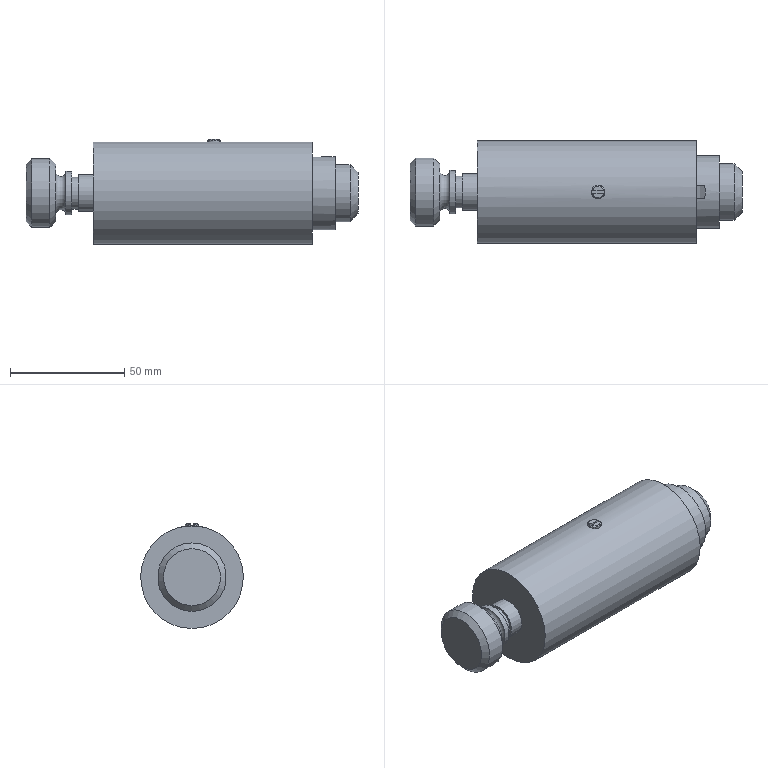Assembly | NX | mm | 5 component files | 5 solids | 56 faces | box 145.41 x 45 x 46 mm | volume 144608 mm3 | plane 26 | cylinder 19 | cone 8 | torus 3 | commonest cylinder face diameters 16 x4 22 x3 32 x2 45 x1 6 x1 5.795 x1 4 x1 12 x1
Bill of materials:
GB75-85,M6x10 | 1 |  | Slotted Set Screw, Long Dog Point, GB 75-85,M6x10
unnamed part 1 | 1 |  | Short solid stepped cylinder with two coaxial diameters: a larger-diameter section and a smaller-diameter section joined at a square shoulder. Both outer ends are chamfered and both end faces are flat.
unnamed part 2 | 1 |  | Straight thin-walled cylindrical tube with plain square-cut ends, a constant outside and inside diameter, and one small round radial hole through the wall at about mid-length.
unnamed part 3 | 1 |  | Turned, stepped pin with an enlarged cylindrical head chamfered on both edges. Next to the head is a rounded-bottom circumferential groove, then a narrow collar and a short small step. Further along are a main cylindrical shank, a reduced-diameter neck, and an end section about the same diameter as the shank, with a small chamfer at the tip.
unnamed part 4 | 1 |  | Straight cylindrical tube with plain ends and one straight longitudinal slot or groove on the outer surface, parallel to the axis. The slot is open at one end and stops short of the other end.
Mates:
1. fix | Fixed_Sleeve 1 component
2. concentric | Top_Block 1 edge | Sliding_Sleeve 1 edge
3. touch align | Sliding_Sleeve 1 face | Screw_Rod 1 face
4. touch align | Sliding_Sleeve 1 face | Fixed_Sleeve 1 face
5. distance | Top_Block 1 face | Fixed_Sleeve 1 face
6. touch align | Set_Screw 1 face | Sliding_Sleeve 1 face
7. touch align | Set_Screw 1 face | Fixed_Sleeve 1 face